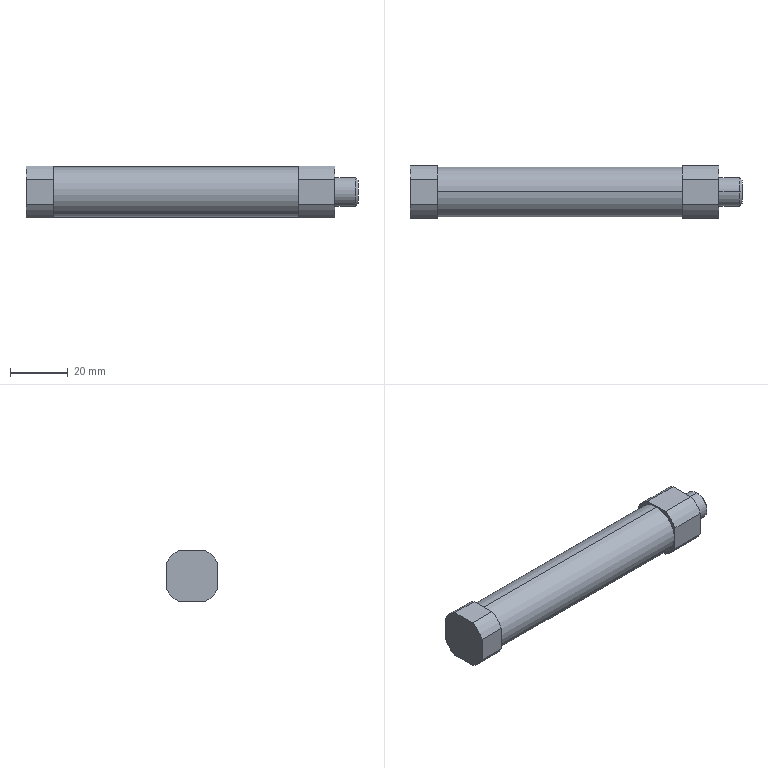Component | SolidWorks | A_CDJ2B16_60_B_0-1_CopyBody_A_CDJ2B16_60_B_0-1 | 1 solid | 40 faces | box 115 x 18 x 18 mm | volume 25719 mm3 | cylinder 18 | plane 16 | cone 6 | commonest cylinder face diameters 20 x8 4.13 x4 5.4 x2 17.4 x2 10 x2
STEP:
#1=COLOUR_RGB('',0.7922,0.8196,0.9333);
#2=FILL_AREA_STYLE_COLOUR('',#1);
#3=FILL_AREA_STYLE('',(#2));
#4=SURFACE_STYLE_FILL_AREA(#3);
#5=SURFACE_SIDE_STYLE('',(#4));
#6=SURFACE_STYLE_USAGE(.BOTH.,#5);
#7=PRESENTATION_STYLE_ASSIGNMENT((#6));
#8=CARTESIAN_POINT('',(-0.6587,0.8964,3.289));
#9=VERTEX_POINT('',#8);
#10=CARTESIAN_POINT('',(-0.6587,0.8964,3.076));
#11=VERTEX_POINT('',#10);
#12=CARTESIAN_POINT('',(-0.6587,0.8964,3.182));
#13=DIRECTION('',(1.,0.,0.));
#14=DIRECTION('',(0.,0.,-1.));
#15=AXIS2_PLACEMENT_3D('',#12,#13,#14);
#16=CIRCLE('',#15,0.1063);
#17=EDGE_CURVE('',#9,#11,#16,.T.);
#18=ORIENTED_EDGE('',*,*,#17,.F.);
#19=CARTESIAN_POINT('',(1.782,0.8964,3.289));
#20=VERTEX_POINT('',#19);
#21=CARTESIAN_POINT('',(-0.6587,0.8964,3.289));
#22=DIRECTION('',(1.,0.,0.));
#23=VECTOR('',#22,39.37);
#24=LINE('',#21,#23);
#25=EDGE_CURVE('',#9,#20,#24,.T.);
#26=ORIENTED_EDGE('',*,*,#25,.T.);
#27=CARTESIAN_POINT('',(1.782,0.8964,3.076));
#28=VERTEX_POINT('',#27);
#29=CARTESIAN_POINT('',(1.782,0.8964,3.182));
#30=DIRECTION('',(1.,0.,0.));
#31=DIRECTION('',(0.,0.,-1.));
#32=AXIS2_PLACEMENT_3D('',#29,#30,#31);
#33=CIRCLE('',#32,0.1063);
#34=EDGE_CURVE('',#20,#28,#33,.T.);
#35=ORIENTED_EDGE('',*,*,#34,.T.);
#36=CARTESIAN_POINT('',(-0.6587,0.8964,3.076));
#37=DIRECTION('',(1.,0.,0.));
#38=VECTOR('',#37,39.37);
#39=LINE('',#36,#38);
#40=EDGE_CURVE('',#11,#28,#39,.T.);
#41=ORIENTED_EDGE('',*,*,#40,.F.);
#42=EDGE_LOOP('',(#18,#26,#35,#41));
#43=FACE_OUTER_BOUND('',#42,.T.);
#44=CARTESIAN_POINT('',(-0.6587,0.8964,3.182));
#45=DIRECTION('',(1.,0.,0.));
#46=DIRECTION('',(0.,0.,-1.));
#47=AXIS2_PLACEMENT_3D('',#44,#45,#46);
#48=CYLINDRICAL_SURFACE('',#47,0.1063);
#49=ADVANCED_FACE('',(#43),#48,.F.);
#50=CARTESIAN_POINT('',(-2.63,1.133,3.182));
#51=VERTEX_POINT('',#50);
#52=CARTESIAN_POINT('',(-2.467,1.133,3.182));
#53=VERTEX_POINT('',#52);
#54=CARTESIAN_POINT('',(-2.548,1.133,3.182));
#55=DIRECTION('',(-0.,1.,-0.));
#56=DIRECTION('',(1.,0.,0.));
#57=AXIS2_PLACEMENT_3D('',#54,#55,#56);
#58=CIRCLE('',#57,0.0813);
#59=EDGE_CURVE('',#51,#53,#58,.T.);
#60=ORIENTED_EDGE('',*,*,#59,.F.);
#61=CARTESIAN_POINT('',(-2.63,1.231,3.182));
#62=VERTEX_POINT('',#61);
#63=CARTESIAN_POINT('',(-2.63,1.133,3.182));
#64=DIRECTION('',(-0.,1.,-0.));
#65=VECTOR('',#64,39.37);
#66=LINE('',#63,#65);
#67=EDGE_CURVE('',#51,#62,#66,.T.);
#68=ORIENTED_EDGE('',*,*,#67,.T.);
#69=CARTESIAN_POINT('',(-2.467,1.231,3.182));
#70=VERTEX_POINT('',#69);
#71=CARTESIAN_POINT('',(-2.548,1.231,3.182));
#72=DIRECTION('',(-0.,1.,-0.));
#73=DIRECTION('',(1.,0.,0.));
#74=AXIS2_PLACEMENT_3D('',#71,#72,#73);
#75=CIRCLE('',#74,0.0813);
#76=EDGE_CURVE('',#62,#70,#75,.T.);
#77=ORIENTED_EDGE('',*,*,#76,.T.);
#78=CARTESIAN_POINT('',(-2.467,1.133,3.182));
#79=DIRECTION('',(-0.,1.,-0.));
#80=VECTOR('',#79,39.37);
#81=LINE('',#78,#80);
#82=EDGE_CURVE('',#53,#70,#81,.T.);
#83=ORIENTED_EDGE('',*,*,#82,.F.);
#84=EDGE_LOOP('',(#60,#68,#77,#83));
#85=FACE_OUTER_BOUND('',#84,.T.);
#86=CARTESIAN_POINT('',(-2.548,1.133,3.182));
#87=DIRECTION('',(-0.,1.,-0.));
#88=DIRECTION('',(1.,0.,0.));
#89=AXIS2_PLACEMENT_3D('',#86,#87,#88);
#90=CYLINDRICAL_SURFACE('',#89,0.0813);
#91=ADVANCED_FACE('',(#85),#90,.F.);
#92=ORIENTED_EDGE('',*,*,#76,.F.);
#93=CARTESIAN_POINT('',(-2.649,1.251,3.182));
#94=VERTEX_POINT('',#93);
#95=CARTESIAN_POINT('',(-2.63,1.231,3.182));
#96=DIRECTION('',(-0.7071,0.7071,-0.));
#97=VECTOR('',#96,39.37);
#98=LINE('',#95,#97);
#99=EDGE_CURVE('',#62,#94,#98,.T.);
#100=ORIENTED_EDGE('',*,*,#99,.T.);
#101=CARTESIAN_POINT('',(-2.447,1.251,3.182));
#102=VERTEX_POINT('',#101);
#103=CARTESIAN_POINT('',(-2.548,1.251,3.182));
#104=DIRECTION('',(-0.,1.,-0.));
#105=DIRECTION('',(-1.,0.,0.));
#106=AXIS2_PLACEMENT_3D('',#103,#104,#105);
#107=CIRCLE('',#106,0.101);
#108=EDGE_CURVE('',#94,#102,#107,.T.);
#109=ORIENTED_EDGE('',*,*,#108,.T.);
#110=CARTESIAN_POINT('',(-2.467,1.231,3.182));
#111=DIRECTION('',(0.7071,0.7071,0.));
#112=VECTOR('',#111,39.37);
#113=LINE('',#110,#112);
#114=EDGE_CURVE('',#70,#102,#113,.T.);
#115=ORIENTED_EDGE('',*,*,#114,.F.);
#116=EDGE_LOOP('',(#92,#100,#109,#115));
#117=FACE_OUTER_BOUND('',#116,.T.);
#118=CARTESIAN_POINT('',(-2.548,1.231,3.182));
#119=DIRECTION('',(-0.,1.,-0.));
#120=DIRECTION('',(1.,0.,0.));
#121=AXIS2_PLACEMENT_3D('',#118,#119,#120);
#122=CONICAL_SURFACE('',#121,0.0813,0.7854);
#123=ADVANCED_FACE('',(#117),#122,.F.);
#124=CARTESIAN_POINT('',(1.071,1.133,3.182));
#125=VERTEX_POINT('',#124);
#126=CARTESIAN_POINT('',(1.234,1.133,3.182));
#127=VERTEX_POINT('',#126);
#128=CARTESIAN_POINT('',(1.152,1.133,3.182));
#129=DIRECTION('',(-0.,1.,-0.));
#130=DIRECTION('',(1.,0.,0.));
#131=AXIS2_PLACEMENT_3D('',#128,#129,#130);
#132=CIRCLE('',#131,0.0813);
#133=EDGE_CURVE('',#125,#127,#132,.T.);
#134=ORIENTED_EDGE('',*,*,#133,.F.);
#135=CARTESIAN_POINT('',(1.071,1.231,3.182));
#136=VERTEX_POINT('',#135);
#137=CARTESIAN_POINT('',(1.071,1.133,3.182));
#138=DIRECTION('',(-0.,1.,-0.));
#139=VECTOR('',#138,39.37);
#140=LINE('',#137,#139);
#141=EDGE_CURVE('',#125,#136,#140,.T.);
#142=ORIENTED_EDGE('',*,*,#141,.T.);
#143=CARTESIAN_POINT('',(1.234,1.231,3.182));
#144=VERTEX_POINT('',#143);
#145=CARTESIAN_POINT('',(1.152,1.231,3.182));
#146=DIRECTION('',(-0.,1.,-0.));
#147=DIRECTION('',(1.,0.,0.));
#148=AXIS2_PLACEMENT_3D('',#145,#146,#147);
#149=CIRCLE('',#148,0.0813);
#150=EDGE_CURVE('',#136,#144,#149,.T.);
#151=ORIENTED_EDGE('',*,*,#150,.T.);
#152=CARTESIAN_POINT('',(1.234,1.133,3.182));
#153=DIRECTION('',(-0.,1.,-0.));
#154=VECTOR('',#153,39.37);
#155=LINE('',#152,#154);
#156=EDGE_CURVE('',#127,#144,#155,.T.);
#157=ORIENTED_EDGE('',*,*,#156,.F.);
#158=EDGE_LOOP('',(#134,#142,#151,#157));
#159=FACE_OUTER_BOUND('',#158,.T.);
#160=CARTESIAN_POINT('',(1.152,1.133,3.182));
#161=DIRECTION('',(-0.,1.,-0.));
#162=DIRECTION('',(1.,0.,0.));
#163=AXIS2_PLACEMENT_3D('',#160,#161,#162);
#164=CYLINDRICAL_SURFACE('',#163,0.0813);
#165=ADVANCED_FACE('',(#159),#164,.F.);
#166=ORIENTED_EDGE('',*,*,#150,.F.);
#167=CARTESIAN_POINT('',(1.051,1.251,3.182));
#168=VERTEX_POINT('',#167);
#169=CARTESIAN_POINT('',(1.071,1.231,3.182));
#170=DIRECTION('',(-0.7071,0.7071,-0.));
#171=VECTOR('',#170,39.37);
#172=LINE('',#169,#171);
#173=EDGE_CURVE('',#136,#168,#172,.T.);
#174=ORIENTED_EDGE('',*,*,#173,.T.);
#175=CARTESIAN_POINT('',(1.253,1.251,3.182));
#176=VERTEX_POINT('',#175);
#177=CARTESIAN_POINT('',(1.152,1.251,3.182));
#178=DIRECTION('',(0.,-1.,0.));
#179=DIRECTION('',(1.,0.,0.));
#180=AXIS2_PLACEMENT_3D('',#177,#178,#179);
#181=CIRCLE('',#180,0.101);
#182=EDGE_CURVE('',#176,#168,#181,.T.);
#183=ORIENTED_EDGE('',*,*,#182,.F.);
#184=CARTESIAN_POINT('',(1.234,1.231,3.182));
#185=DIRECTION('',(0.7071,0.7071,0.));
#186=VECTOR('',#185,39.37);
#187=LINE('',#184,#186);
#188=EDGE_CURVE('',#144,#176,#187,.T.);
#189=ORIENTED_EDGE('',*,*,#188,.F.);
#190=EDGE_LOOP('',(#166,#174,#183,#189));
#191=FACE_OUTER_BOUND('',#190,.T.);
#192=CARTESIAN_POINT('',(1.152,1.231,3.182));
#193=DIRECTION('',(-0.,1.,-0.));
#194=DIRECTION('',(1.,0.,0.));
#195=AXIS2_PLACEMENT_3D('',#192,#193,#194);
#196=CONICAL_SURFACE('',#195,0.0813,0.7854);
#197=ADVANCED_FACE('',(#191),#196,.F.);
#198=CARTESIAN_POINT('',(-2.371,0.8964,2.84));
#199=VERTEX_POINT('',#198);
#200=CARTESIAN_POINT('',(-2.371,0.8964,3.525));
#201=VERTEX_POINT('',#200);
#202=CARTESIAN_POINT('',(-2.371,0.8964,3.182));
#203=DIRECTION('',(1.,0.,0.));
#204=DIRECTION('',(0.,0.,-1.));
#205=AXIS2_PLACEMENT_3D('',#202,#203,#204);
#206=CIRCLE('',#205,0.3425);
#207=EDGE_CURVE('',#199,#201,#206,.T.);
#208=ORIENTED_EDGE('',*,*,#207,.T.);
#209=CARTESIAN_POINT('',(0.9752,0.8964,3.525));
#210=VERTEX_POINT('',#209);
#211=CARTESIAN_POINT('',(-2.735,0.8964,3.525));
#212=DIRECTION('',(1.,0.,0.));
#213=VECTOR('',#212,39.37);
#214=LINE('',#211,#213);
#215=EDGE_CURVE('',#201,#210,#214,.T.);
#216=ORIENTED_EDGE('',*,*,#215,.T.);
#217=CARTESIAN_POINT('',(0.9752,0.8964,2.84));
#218=VERTEX_POINT('',#217);
#219=CARTESIAN_POINT('',(0.9752,0.8964,3.182));
#220=DIRECTION('',(1.,0.,0.));
#221=DIRECTION('',(0.,0.,-1.));
#222=AXIS2_PLACEMENT_3D('',#219,#220,#221);
#223=CIRCLE('',#222,0.3425);
#224=EDGE_CURVE('',#218,#210,#223,.T.);
#225=ORIENTED_EDGE('',*,*,#224,.F.);
#226=CARTESIAN_POINT('',(-2.735,0.8964,2.84));
#227=DIRECTION('',(1.,0.,0.));
#228=VECTOR('',#227,39.37);
#229=LINE('',#226,#228);
#230=EDGE_CURVE('',#199,#218,#229,.T.);
#231=ORIENTED_EDGE('',*,*,#230,.F.);
#232=EDGE_LOOP('',(#208,#216,#225,#231));
#233=FACE_OUTER_BOUND('',#232,.T.);
#234=CARTESIAN_POINT('',(-2.735,0.8964,3.182));
#235=DIRECTION('',(1.,0.,0.));
#236=DIRECTION('',(0.,0.,-1.));
#237=AXIS2_PLACEMENT_3D('',#234,#235,#236);
#238=CYLINDRICAL_SURFACE('',#237,0.3425);
#239=ADVANCED_FACE('',(#233),#238,.T.);
#240=CARTESIAN_POINT('',(1.467,0.8964,2.985));
#241=VERTEX_POINT('',#240);
#242=CARTESIAN_POINT('',(1.467,0.8964,3.379));
#243=VERTEX_POINT('',#242);
#244=CARTESIAN_POINT('',(1.467,0.8964,3.182));
#245=DIRECTION('',(1.,0.,0.));
#246=DIRECTION('',(0.,0.,-1.));
#247=AXIS2_PLACEMENT_3D('',#244,#245,#246);
#248=CIRCLE('',#247,0.1969);
#249=EDGE_CURVE('',#241,#243,#248,.T.);
#250=ORIENTED_EDGE('',*,*,#249,.T.);
#251=CARTESIAN_POINT('',(1.746,0.8964,3.379));
#252=VERTEX_POINT('',#251);
#253=CARTESIAN_POINT('',(-2.735,0.8964,3.379));
#254=DIRECTION('',(1.,0.,0.));
#255=VECTOR('',#254,39.37);
#256=LINE('',#253,#255);
#257=EDGE_CURVE('',#243,#252,#256,.T.);
#258=ORIENTED_EDGE('',*,*,#257,.T.);
#259=CARTESIAN_POINT('',(1.746,0.8964,2.985));
#260=VERTEX_POINT('',#259);
#261=CARTESIAN_POINT('',(1.746,0.8964,3.182));
#262=DIRECTION('',(1.,0.,0.));
#263=DIRECTION('',(0.,0.,-1.));
#264=AXIS2_PLACEMENT_3D('',#261,#262,#263);
#265=CIRCLE('',#264,0.1969);
#266=EDGE_CURVE('',#260,#252,#265,.T.);
#267=ORIENTED_EDGE('',*,*,#266,.F.);
#268=CARTESIAN_POINT('',(-2.735,0.8964,2.985));
#269=DIRECTION('',(1.,0.,0.));
#270=VECTOR('',#269,39.37);
#271=LINE('',#268,#270);
#272=EDGE_CURVE('',#241,#260,#271,.T.);
#273=ORIENTED_EDGE('',*,*,#272,.F.);
#274=EDGE_LOOP('',(#250,#258,#267,#273));
#275=FACE_OUTER_BOUND('',#274,.T.);
#276=CARTESIAN_POINT('',(-2.735,0.8964,3.182));
#277=DIRECTION('',(1.,0.,0.));
#278=DIRECTION('',(0.,0.,-1.));
#279=AXIS2_PLACEMENT_3D('',#276,#277,#278);
#280=CYLINDRICAL_SURFACE('',#279,0.1969);
#281=ADVANCED_FACE('',(#275),#280,.T.);
#282=CARTESIAN_POINT('',(1.782,0.8964,3.022));
#283=VERTEX_POINT('',#282);
#284=CARTESIAN_POINT('',(1.782,0.8964,3.343));
#285=VERTEX_POINT('',#284);
#286=CARTESIAN_POINT('',(1.782,0.8964,3.182));
#287=DIRECTION('',(1.,0.,0.));
#288=DIRECTION('',(0.,0.,-1.));
#289=AXIS2_PLACEMENT_3D('',#286,#287,#288);
#290=CIRCLE('',#289,0.1606);
#291=EDGE_CURVE('',#283,#285,#290,.T.);
#292=ORIENTED_EDGE('',*,*,#291,.F.);
#293=CARTESIAN_POINT('',(1.746,0.8964,2.985));
#294=DIRECTION('',(-0.7071,0.,-0.7071));
#295=VECTOR('',#294,39.37);
#296=LINE('',#293,#295);
#297=EDGE_CURVE('',#283,#260,#296,.T.);
#298=ORIENTED_EDGE('',*,*,#297,.T.);
#299=ORIENTED_EDGE('',*,*,#266,.T.);
#300=CARTESIAN_POINT('',(1.746,0.8964,3.379));
#301=DIRECTION('',(-0.7071,-0.,0.7071));
#302=VECTOR('',#301,39.37);
#303=LINE('',#300,#302);
#304=EDGE_CURVE('',#285,#252,#303,.T.);
#305=ORIENTED_EDGE('',*,*,#304,.F.);
#306=EDGE_LOOP('',(#292,#298,#299,#305));
#307=FACE_OUTER_BOUND('',#306,.T.);
#308=CARTESIAN_POINT('',(1.746,0.8964,3.182));
#309=DIRECTION('',(-1.,-0.,-0.));
#310=DIRECTION('',(0.,0.,1.));
#311=AXIS2_PLACEMENT_3D('',#308,#309,#310);
#312=CONICAL_SURFACE('',#311,0.1969,0.7854);
#313=ADVANCED_FACE('',(#307),#312,.T.);
#314=CARTESIAN_POINT('',(-2.745,1.251,3.011));
#315=VERTEX_POINT('',#314);
#316=CARTESIAN_POINT('',(-2.745,1.251,3.354));
#317=VERTEX_POINT('',#316);
#318=CARTESIAN_POINT('',(-2.745,1.251,3.011));
#319=DIRECTION('',(-0.,0.,1.));
#320=VECTOR('',#319,39.37);
#321=LINE('',#318,#320);
#322=EDGE_CURVE('',#315,#317,#321,.T.);
#323=ORIENTED_EDGE('',*,*,#322,.T.);
#324=CARTESIAN_POINT('',(-2.371,1.251,3.354));
#325=VERTEX_POINT('',#324);
#326=CARTESIAN_POINT('',(-2.371,1.251,3.354));
#327=DIRECTION('',(-1.,-0.,-0.));
#328=VECTOR('',#327,39.37);
#329=LINE('',#326,#328);
#330=EDGE_CURVE('',#325,#317,#329,.T.);
#331=ORIENTED_EDGE('',*,*,#330,.F.);
#332=CARTESIAN_POINT('',(-2.371,1.251,3.011));
#333=VERTEX_POINT('',#332);
#334=CARTESIAN_POINT('',(-2.371,1.251,3.011));
#335=DIRECTION('',(-0.,0.,1.));
#336=VECTOR('',#335,39.37);
#337=LINE('',#334,#336);
#338=EDGE_CURVE('',#333,#325,#337,.T.);
#339=ORIENTED_EDGE('',*,*,#338,.F.);
#340=CARTESIAN_POINT('',(-2.371,1.251,3.011));
#341=DIRECTION('',(-1.,-0.,-0.));
#342=VECTOR('',#341,39.37);
#343=LINE('',#340,#342);
#344=EDGE_CURVE('',#333,#315,#343,.T.);
#345=ORIENTED_EDGE('',*,*,#344,.T.);
#346=EDGE_LOOP('',(#323,#331,#339,#345));
#347=FACE_OUTER_BOUND('',#346,.T.);
#348=CARTESIAN_POINT('',(-2.548,1.251,3.182));
#349=DIRECTION('',(-0.,1.,-0.));
#350=DIRECTION('',(-1.,0.,0.));
#351=AXIS2_PLACEMENT_3D('',#348,#349,#350);
#352=CIRCLE('',#351,0.101);
#353=EDGE_CURVE('',#102,#94,#352,.T.);
#354=ORIENTED_EDGE('',*,*,#353,.F.);
#355=ORIENTED_EDGE('',*,*,#108,.F.);
#356=EDGE_LOOP('',(#354,#355));
#357=FACE_BOUND('',#356,.T.);
#358=CARTESIAN_POINT('',(-2.371,1.251,3.011));
#359=DIRECTION('',(0.,-1.,0.));
#360=DIRECTION('',(-1.,-0.,-0.));
#361=AXIS2_PLACEMENT_3D('',#358,#359,#360);
#362=PLANE('',#361);
#363=ADVANCED_FACE('',(#347,#357),#362,.F.);
#364=CARTESIAN_POINT('',(1.467,1.251,3.011));
#365=VERTEX_POINT('',#364);
#366=CARTESIAN_POINT('',(1.467,1.251,3.354));
#367=VERTEX_POINT('',#366);
#368=CARTESIAN_POINT('',(1.467,1.251,3.011));
#369=DIRECTION('',(-0.,0.,1.));
#370=VECTOR('',#369,39.37);
#371=LINE('',#368,#370);
#372=EDGE_CURVE('',#365,#367,#371,.T.);
#373=ORIENTED_EDGE('',*,*,#372,.F.);
#374=CARTESIAN_POINT('',(0.9752,1.251,3.011));
#375=VERTEX_POINT('',#374);
#376=CARTESIAN_POINT('',(0.9752,1.251,3.011));
#377=DIRECTION('',(1.,0.,0.));
#378=VECTOR('',#377,39.37);
#379=LINE('',#376,#378);
#380=EDGE_CURVE('',#375,#365,#379,.T.);
#381=ORIENTED_EDGE('',*,*,#380,.F.);
#382=CARTESIAN_POINT('',(0.9752,1.251,3.354));
#383=VERTEX_POINT('',#382);
#384=CARTESIAN_POINT('',(0.9752,1.251,3.011));
#385=DIRECTION('',(-0.,0.,1.));
#386=VECTOR('',#385,39.37);
#387=LINE('',#384,#386);
#388=EDGE_CURVE('',#375,#383,#387,.T.);
#389=ORIENTED_EDGE('',*,*,#388,.T.);
#390=CARTESIAN_POINT('',(0.9752,1.251,3.354));
#391=DIRECTION('',(1.,0.,0.));
#392=VECTOR('',#391,39.37);
#393=LINE('',#390,#392);
#394=EDGE_CURVE('',#383,#367,#393,.T.);
#395=ORIENTED_EDGE('',*,*,#394,.T.);
#396=EDGE_LOOP('',(#373,#381,#389,#395));
#397=FACE_OUTER_BOUND('',#396,.T.);
#398=ORIENTED_EDGE('',*,*,#182,.T.);
#399=CARTESIAN_POINT('',(1.152,1.251,3.182));
#400=DIRECTION('',(0.,-1.,0.));
#401=DIRECTION('',(1.,0.,0.));
#402=AXIS2_PLACEMENT_3D('',#399,#400,#401);
#403=CIRCLE('',#402,0.101);
#404=EDGE_CURVE('',#168,#176,#403,.T.);
#405=ORIENTED_EDGE('',*,*,#404,.T.);
#406=EDGE_LOOP('',(#398,#405));
#407=FACE_BOUND('',#406,.T.);
#408=CARTESIAN_POINT('',(0.9752,1.251,3.011));
#409=DIRECTION('',(-0.,1.,-0.));
#410=DIRECTION('',(1.,0.,0.));
#411=AXIS2_PLACEMENT_3D('',#408,#409,#410);
#412=PLANE('',#411);
#413=ADVANCED_FACE('',(#397,#407),#412,.T.);
#414=CARTESIAN_POINT('',(1.782,0.8964,3.182));
#415=DIRECTION('',(1.,0.,0.));
#416=DIRECTION('',(0.,0.,-1.));
#417=AXIS2_PLACEMENT_3D('',#414,#415,#416);
#418=CIRCLE('',#417,0.1063);
#419=EDGE_CURVE('',#28,#20,#418,.T.);
#420=ORIENTED_EDGE('',*,*,#419,.F.);
#421=ORIENTED_EDGE('',*,*,#34,.F.);
#422=EDGE_LOOP('',(#420,#421));
#423=FACE_BOUND('',#422,.T.);
#424=CARTESIAN_POINT('',(1.782,0.8964,3.182));
#425=DIRECTION('',(1.,0.,0.));
#426=DIRECTION('',(0.,0.,-1.));
#427=AXIS2_PLACEMENT_3D('',#424,#425,#426);
#428=CIRCLE('',#427,0.1606);
#429=EDGE_CURVE('',#285,#283,#428,.T.);
#430=ORIENTED_EDGE('',*,*,#429,.T.);
#431=ORIENTED_EDGE('',*,*,#291,.T.);
#432=EDGE_LOOP('',(#430,#431));
#433=FACE_OUTER_BOUND('',#432,.T.);
#434=CARTESIAN_POINT('',(1.782,0.8964,3.182));
#435=DIRECTION('',(-1.,-0.,-0.));
#436=DIRECTION('',(-0.,0.,1.));
#437=AXIS2_PLACEMENT_3D('',#434,#435,#436);
#438=PLANE('',#437);
#439=ADVANCED_FACE('',(#423,#433),#438,.F.);
#440=ORIENTED_EDGE('',*,*,#297,.F.);
#441=ORIENTED_EDGE('',*,*,#429,.F.);
#442=ORIENTED_EDGE('',*,*,#304,.T.);
#443=CARTESIAN_POINT('',(1.746,0.8964,3.182));
#444=DIRECTION('',(1.,0.,0.));
#445=DIRECTION('',(0.,0.,-1.));
#446=AXIS2_PLACEMENT_3D('',#443,#444,#445);
#447=CIRCLE('',#446,0.1969);
#448=EDGE_CURVE('',#252,#260,#447,.T.);
#449=ORIENTED_EDGE('',*,*,#448,.T.);
#450=EDGE_LOOP('',(#440,#441,#442,#449));
#451=FACE_OUTER_BOUND('',#450,.T.);
#452=CARTESIAN_POINT('',(1.746,0.8964,3.182));
#453=DIRECTION('',(-1.,-0.,-0.));
#454=DIRECTION('',(0.,0.,1.));
#455=AXIS2_PLACEMENT_3D('',#452,#453,#454);
#456=CONICAL_SURFACE('',#455,0.1969,0.7854);
#457=ADVANCED_FACE('',(#451),#456,.T.);
#458=ORIENTED_EDGE('',*,*,#257,.F.);
#459=CARTESIAN_POINT('',(1.467,0.8964,3.182));
#460=DIRECTION('',(1.,0.,0.));
#461=DIRECTION('',(0.,0.,-1.));
#462=AXIS2_PLACEMENT_3D('',#459,#460,#461);
#463=CIRCLE('',#462,0.1969);
#464=EDGE_CURVE('',#243,#241,#463,.T.);
#465=ORIENTED_EDGE('',*,*,#464,.T.);
#466=ORIENTED_EDGE('',*,*,#272,.T.);
#467=ORIENTED_EDGE('',*,*,#448,.F.);
#468=EDGE_LOOP('',(#458,#465,#466,#467));
#469=FACE_OUTER_BOUND('',#468,.T.);
#470=CARTESIAN_POINT('',(-2.735,0.8964,3.182));
#471=DIRECTION('',(1.,0.,0.));
#472=DIRECTION('',(0.,0.,-1.));
#473=AXIS2_PLACEMENT_3D('',#470,#471,#472);
#474=CYLINDRICAL_SURFACE('',#473,0.1969);
#475=ADVANCED_FACE('',(#469),#474,.T.);
#476=CARTESIAN_POINT('',(1.467,0.7248,3.537));
#477=VERTEX_POINT('',#476);
#478=CARTESIAN_POINT('',(1.467,0.5421,3.354));
#479=VERTEX_POINT('',#478);
#480=CARTESIAN_POINT('',(1.467,0.8964,3.182));
#481=DIRECTION('',(1.,0.,0.));
#482=DIRECTION('',(0.,0.,-1.));
#483=AXIS2_PLACEMENT_3D('',#480,#481,#482);
#484=CIRCLE('',#483,0.3937);
#485=EDGE_CURVE('',#477,#479,#484,.T.);
#486=ORIENTED_EDGE('',*,*,#485,.T.);
#487=CARTESIAN_POINT('',(1.467,0.5421,3.011));
#488=VERTEX_POINT('',#487);
#489=CARTESIAN_POINT('',(1.467,0.5421,3.354));
#490=DIRECTION('',(0.,-0.,-1.));
#491=VECTOR('',#490,39.37);
#492=LINE('',#489,#491);
#493=EDGE_CURVE('',#479,#488,#492,.T.);
#494=ORIENTED_EDGE('',*,*,#493,.T.);
#495=CARTESIAN_POINT('',(1.467,0.7248,2.828));
#496=VERTEX_POINT('',#495);
#497=CARTESIAN_POINT('',(1.467,0.8964,3.182));
#498=DIRECTION('',(1.,0.,0.));
#499=DIRECTION('',(0.,0.,-1.));
#500=AXIS2_PLACEMENT_3D('',#497,#498,#499);
#501=CIRCLE('',#500,0.3937);
#502=EDGE_CURVE('',#488,#496,#501,.T.);
#503=ORIENTED_EDGE('',*,*,#502,.T.);
#504=CARTESIAN_POINT('',(1.467,1.068,2.828));
#505=VERTEX_POINT('',#504);
#506=CARTESIAN_POINT('',(1.467,0.7248,2.828));
#507=DIRECTION('',(-0.,1.,-0.));
#508=VECTOR('',#507,39.37);
#509=LINE('',#506,#508);
#510=EDGE_CURVE('',#496,#505,#509,.T.);
#511=ORIENTED_EDGE('',*,*,#510,.T.);
#512=CARTESIAN_POINT('',(1.467,0.8964,3.182));
#513=DIRECTION('',(1.,0.,0.));
#514=DIRECTION('',(0.,0.,-1.));
#515=AXIS2_PLACEMENT_3D('',#512,#513,#514);
#516=CIRCLE('',#515,0.3937);
#517=EDGE_CURVE('',#505,#365,#516,.T.);
#518=ORIENTED_EDGE('',*,*,#517,.T.);
#519=ORIENTED_EDGE('',*,*,#372,.T.);
#520=CARTESIAN_POINT('',(1.467,1.068,3.537));
#521=VERTEX_POINT('',#520);
#522=CARTESIAN_POINT('',(1.467,0.8964,3.182));
#523=DIRECTION('',(1.,0.,0.));
#524=DIRECTION('',(0.,0.,-1.));
#525=AXIS2_PLACEMENT_3D('',#522,#523,#524);
#526=CIRCLE('',#525,0.3937);
#527=EDGE_CURVE('',#367,#521,#526,.T.);
#528=ORIENTED_EDGE('',*,*,#527,.T.);
#529=CARTESIAN_POINT('',(1.467,1.068,3.537));
#530=DIRECTION('',(0.,-1.,0.));
#531=VECTOR('',#530,39.37);
#532=LINE('',#529,#531);
#533=EDGE_CURVE('',#521,#477,#532,.T.);
#534=ORIENTED_EDGE('',*,*,#533,.T.);
#535=EDGE_LOOP('',(#486,#494,#503,#511,#518,#519,#528,#534));
#536=FACE_OUTER_BOUND('',#535,.T.);
#537=ORIENTED_EDGE('',*,*,#249,.F.);
#538=ORIENTED_EDGE('',*,*,#464,.F.);
#539=EDGE_LOOP('',(#537,#538));
#540=FACE_BOUND('',#539,.T.);
#541=CARTESIAN_POINT('',(1.467,0.8964,3.182));
#542=DIRECTION('',(1.,0.,0.));
#543=DIRECTION('',(0.,-0.,-1.));
#544=AXIS2_PLACEMENT_3D('',#541,#542,#543);
#545=PLANE('',#544);
#546=ADVANCED_FACE('',(#536,#540),#545,.T.);
#547=CARTESIAN_POINT('',(0.9752,0.7248,3.537));
#548=VERTEX_POINT('',#547);
#549=CARTESIAN_POINT('',(0.9752,0.5421,3.354));
#550=VERTEX_POINT('',#549);
#551=CARTESIAN_POINT('',(0.9752,0.8964,3.182));
#552=DIRECTION('',(1.,0.,0.));
#553=DIRECTION('',(0.,0.,-1.));
#554=AXIS2_PLACEMENT_3D('',#551,#552,#553);
#555=CIRCLE('',#554,0.3937);
#556=EDGE_CURVE('',#548,#550,#555,.T.);
#557=ORIENTED_EDGE('',*,*,#556,.F.);
#558=CARTESIAN_POINT('',(0.9752,1.068,3.537));
#559=VERTEX_POINT('',#558);
#560=CARTESIAN_POINT('',(0.9752,1.068,3.537));
#561=DIRECTION('',(0.,-1.,0.));
#562=VECTOR('',#561,39.37);
#563=LINE('',#560,#562);
#564=EDGE_CURVE('',#559,#548,#563,.T.);
#565=ORIENTED_EDGE('',*,*,#564,.F.);
#566=CARTESIAN_POINT('',(0.9752,0.8964,3.182));
#567=DIRECTION('',(1.,0.,0.));
#568=DIRECTION('',(0.,0.,-1.));
#569=AXIS2_PLACEMENT_3D('',#566,#567,#568);
#570=CIRCLE('',#569,0.3937);
#571=EDGE_CURVE('',#383,#559,#570,.T.);
#572=ORIENTED_EDGE('',*,*,#571,.F.);
#573=ORIENTED_EDGE('',*,*,#388,.F.);
#574=CARTESIAN_POINT('',(0.9752,1.068,2.828));
#575=VERTEX_POINT('',#574);
#576=CARTESIAN_POINT('',(0.9752,0.8964,3.182));
#577=DIRECTION('',(1.,0.,0.));
#578=DIRECTION('',(0.,0.,-1.));
#579=AXIS2_PLACEMENT_3D('',#576,#577,#578);
#580=CIRCLE('',#579,0.3937);
#581=EDGE_CURVE('',#575,#375,#580,.T.);
#582=ORIENTED_EDGE('',*,*,#581,.F.);
#583=CARTESIAN_POINT('',(0.9752,0.7248,2.828));
#584=VERTEX_POINT('',#583);
#585=CARTESIAN_POINT('',(0.9752,0.7248,2.828));
#586=DIRECTION('',(-0.,1.,-0.));
#587=VECTOR('',#586,39.37);
#588=LINE('',#585,#587);
#589=EDGE_CURVE('',#584,#575,#588,.T.);
#590=ORIENTED_EDGE('',*,*,#589,.F.);
#591=CARTESIAN_POINT('',(0.9752,0.5421,3.011));
#592=VERTEX_POINT('',#591);
#593=CARTESIAN_POINT('',(0.9752,0.8964,3.182));
#594=DIRECTION('',(1.,0.,0.));
#595=DIRECTION('',(0.,0.,-1.));
#596=AXIS2_PLACEMENT_3D('',#593,#594,#595);
#597=CIRCLE('',#596,0.3937);
#598=EDGE_CURVE('',#592,#584,#597,.T.);
#599=ORIENTED_EDGE('',*,*,#598,.F.);
#600=CARTESIAN_POINT('',(0.9752,0.5421,3.354));
#601=DIRECTION('',(0.,-0.,-1.));
#602=VECTOR('',#601,39.37);
#603=LINE('',#600,#602);
#604=EDGE_CURVE('',#550,#592,#603,.T.);
#605=ORIENTED_EDGE('',*,*,#604,.F.);
#606=EDGE_LOOP('',(#557,#565,#572,#573,#582,#590,#599,#605));
#607=FACE_OUTER_BOUND('',#606,.T.);
#608=ORIENTED_EDGE('',*,*,#224,.T.);
#609=CARTESIAN_POINT('',(0.9752,0.8964,3.182));
#610=DIRECTION('',(1.,0.,0.));
#611=DIRECTION('',(0.,0.,-1.));
#612=AXIS2_PLACEMENT_3D('',#609,#610,#611);
#613=CIRCLE('',#612,0.3425);
#614=EDGE_CURVE('',#210,#218,#613,.T.);
#615=ORIENTED_EDGE('',*,*,#614,.T.);
#616=EDGE_LOOP('',(#608,#615));
#617=FACE_BOUND('',#616,.T.);
#618=CARTESIAN_POINT('',(0.9752,0.8964,3.182));
#619=DIRECTION('',(1.,0.,0.));
#620=DIRECTION('',(0.,-0.,-1.));
#621=AXIS2_PLACEMENT_3D('',#618,#619,#620);
#622=PLANE('',#621);
#623=ADVANCED_FACE('',(#607,#617),#622,.F.);
#624=ORIENTED_EDGE('',*,*,#485,.F.);
#625=CARTESIAN_POINT('',(0.9752,0.7248,3.537));
#626=DIRECTION('',(1.,0.,0.));
#627=VECTOR('',#626,39.37);
#628=LINE('',#625,#627);
#629=EDGE_CURVE('',#548,#477,#628,.T.);
#630=ORIENTED_EDGE('',*,*,#629,.F.);
#631=ORIENTED_EDGE('',*,*,#556,.T.);
#632=CARTESIAN_POINT('',(0.9752,0.5421,3.354));
#633=DIRECTION('',(1.,0.,0.));
#634=VECTOR('',#633,39.37);
#635=LINE('',#632,#634);
#636=EDGE_CURVE('',#550,#479,#635,.T.);
#637=ORIENTED_EDGE('',*,*,#636,.T.);
#638=EDGE_LOOP('',(#624,#630,#631,#637));
#639=FACE_OUTER_BOUND('',#638,.T.);
#640=CARTESIAN_POINT('',(0.9752,0.8964,3.182));
#641=DIRECTION('',(1.,0.,0.));
#642=DIRECTION('',(0.,0.,-1.));
#643=AXIS2_PLACEMENT_3D('',#640,#641,#642);
#644=CYLINDRICAL_SURFACE('',#643,0.3937);
#645=ADVANCED_FACE('',(#639),#644,.T.);
#646=ORIENTED_EDGE('',*,*,#533,.F.);
#647=CARTESIAN_POINT('',(0.9752,1.068,3.537));
#648=DIRECTION('',(1.,0.,0.));
#649=VECTOR('',#648,39.37);
#650=LINE('',#647,#649);
#651=EDGE_CURVE('',#559,#521,#650,.T.);
#652=ORIENTED_EDGE('',*,*,#651,.F.);
#653=ORIENTED_EDGE('',*,*,#564,.T.);
#654=ORIENTED_EDGE('',*,*,#629,.T.);
#655=EDGE_LOOP('',(#646,#652,#653,#654));
#656=FACE_OUTER_BOUND('',#655,.T.);
#657=CARTESIAN_POINT('',(0.9752,1.068,3.537));
#658=DIRECTION('',(-0.,0.,1.));
#659=DIRECTION('',(1.,0.,0.));
#660=AXIS2_PLACEMENT_3D('',#657,#658,#659);
#661=PLANE('',#660);
#662=ADVANCED_FACE('',(#656),#661,.T.);
#663=ORIENTED_EDGE('',*,*,#527,.F.);
#664=ORIENTED_EDGE('',*,*,#394,.F.);
#665=ORIENTED_EDGE('',*,*,#571,.T.);
#666=ORIENTED_EDGE('',*,*,#651,.T.);
#667=EDGE_LOOP('',(#663,#664,#665,#666));
#668=FACE_OUTER_BOUND('',#667,.T.);
#669=CARTESIAN_POINT('',(0.9752,0.8964,3.182));
#670=DIRECTION('',(1.,0.,0.));
#671=DIRECTION('',(0.,0.,-1.));
#672=AXIS2_PLACEMENT_3D('',#669,#670,#671);
#673=CYLINDRICAL_SURFACE('',#672,0.3937);
#674=ADVANCED_FACE('',(#668),#673,.T.);
#675=ORIENTED_EDGE('',*,*,#517,.F.);
#676=CARTESIAN_POINT('',(0.9752,1.068,2.828));
#677=DIRECTION('',(1.,0.,0.));
#678=VECTOR('',#677,39.37);
#679=LINE('',#676,#678);
#680=EDGE_CURVE('',#575,#505,#679,.T.);
#681=ORIENTED_EDGE('',*,*,#680,.F.);
#682=ORIENTED_EDGE('',*,*,#581,.T.);
#683=ORIENTED_EDGE('',*,*,#380,.T.);
#684=EDGE_LOOP('',(#675,#681,#682,#683));
#685=FACE_OUTER_BOUND('',#684,.T.);
#686=CARTESIAN_POINT('',(0.9752,0.8964,3.182));
#687=DIRECTION('',(1.,0.,0.));
#688=DIRECTION('',(0.,0.,-1.));
#689=AXIS2_PLACEMENT_3D('',#686,#687,#688);
#690=CYLINDRICAL_SURFACE('',#689,0.3937);
#691=ADVANCED_FACE('',(#685),#690,.T.);
#692=ORIENTED_EDGE('',*,*,#510,.F.);
#693=CARTESIAN_POINT('',(0.9752,0.7248,2.828));
#694=DIRECTION('',(1.,0.,0.));
#695=VECTOR('',#694,39.37);
#696=LINE('',#693,#695);
#697=EDGE_CURVE('',#584,#496,#696,.T.);
#698=ORIENTED_EDGE('',*,*,#697,.F.);
#699=ORIENTED_EDGE('',*,*,#589,.T.);
#700=ORIENTED_EDGE('',*,*,#680,.T.);
#701=EDGE_LOOP('',(#692,#698,#699,#700));
#702=FACE_OUTER_BOUND('',#701,.T.);
#703=CARTESIAN_POINT('',(0.9752,0.7248,2.828));
#704=DIRECTION('',(0.,-0.,-1.));
#705=DIRECTION('',(-1.,-0.,-0.));
#706=AXIS2_PLACEMENT_3D('',#703,#704,#705);
#707=PLANE('',#706);
#708=ADVANCED_FACE('',(#702),#707,.T.);
#709=ORIENTED_EDGE('',*,*,#502,.F.);
#710=CARTESIAN_POINT('',(0.9752,0.5421,3.011));
#711=DIRECTION('',(1.,0.,0.));
#712=VECTOR('',#711,39.37);
#713=LINE('',#710,#712);
#714=EDGE_CURVE('',#592,#488,#713,.T.);
#715=ORIENTED_EDGE('',*,*,#714,.F.);
#716=ORIENTED_EDGE('',*,*,#598,.T.);
#717=ORIENTED_EDGE('',*,*,#697,.T.);
#718=EDGE_LOOP('',(#709,#715,#716,#717));
#719=FACE_OUTER_BOUND('',#718,.T.);
#720=CARTESIAN_POINT('',(0.9752,0.8964,3.182));
#721=DIRECTION('',(1.,0.,0.));
#722=DIRECTION('',(0.,0.,-1.));
#723=AXIS2_PLACEMENT_3D('',#720,#721,#722);
#724=CYLINDRICAL_SURFACE('',#723,0.3937);
#725=ADVANCED_FACE('',(#719),#724,.T.);
#726=ORIENTED_EDGE('',*,*,#493,.F.);
#727=ORIENTED_EDGE('',*,*,#636,.F.);
#728=ORIENTED_EDGE('',*,*,#604,.T.);
#729=ORIENTED_EDGE('',*,*,#714,.T.);
#730=EDGE_LOOP('',(#726,#727,#728,#729));
#731=FACE_OUTER_BOUND('',#730,.T.);
#732=CARTESIAN_POINT('',(0.9752,0.5421,3.354));
#733=DIRECTION('',(0.,-1.,0.));
#734=DIRECTION('',(-1.,-0.,-0.));
#735=AXIS2_PLACEMENT_3D('',#732,#733,#734);
#736=PLANE('',#735);
#737=ADVANCED_FACE('',(#731),#736,.T.);
#738=ORIENTED_EDGE('',*,*,#215,.F.);
#739=CARTESIAN_POINT('',(-2.371,0.8964,3.182));
#740=DIRECTION('',(1.,0.,0.));
#741=DIRECTION('',(0.,0.,-1.));
#742=AXIS2_PLACEMENT_3D('',#739,#740,#741);
#743=CIRCLE('',#742,0.3425);
#744=EDGE_CURVE('',#201,#199,#743,.T.);
#745=ORIENTED_EDGE('',*,*,#744,.T.);
#746=ORIENTED_EDGE('',*,*,#230,.T.);
#747=ORIENTED_EDGE('',*,*,#614,.F.);
#748=EDGE_LOOP('',(#738,#745,#746,#747));
#749=FACE_OUTER_BOUND('',#748,.T.);
#750=CARTESIAN_POINT('',(-2.735,0.8964,3.182));
#751=DIRECTION('',(1.,0.,0.));
#752=DIRECTION('',(0.,0.,-1.));
#753=AXIS2_PLACEMENT_3D('',#750,#751,#752);
#754=CYLINDRICAL_SURFACE('',#753,0.3425);
#755=ADVANCED_FACE('',(#749),#754,.T.);
#756=CARTESIAN_POINT('',(-2.371,0.7248,3.537));
#757=VERTEX_POINT('',#756);
#758=CARTESIAN_POINT('',(-2.371,0.5421,3.354));
#759=VERTEX_POINT('',#758);
#760=CARTESIAN_POINT('',(-2.371,0.8964,3.182));
#761=DIRECTION('',(1.,0.,0.));
#762=DIRECTION('',(0.,0.,-1.));
#763=AXIS2_PLACEMENT_3D('',#760,#761,#762);
#764=CIRCLE('',#763,0.3937);
#765=EDGE_CURVE('',#757,#759,#764,.T.);
#766=ORIENTED_EDGE('',*,*,#765,.T.);
#767=CARTESIAN_POINT('',(-2.371,0.5421,3.011));
#768=VERTEX_POINT('',#767);
#769=CARTESIAN_POINT('',(-2.371,0.5421,3.354));
#770=DIRECTION('',(0.,-0.,-1.));
#771=VECTOR('',#770,39.37);
#772=LINE('',#769,#771);
#773=EDGE_CURVE('',#759,#768,#772,.T.);
#774=ORIENTED_EDGE('',*,*,#773,.T.);
#775=CARTESIAN_POINT('',(-2.371,0.7248,2.828));
#776=VERTEX_POINT('',#775);
#777=CARTESIAN_POINT('',(-2.371,0.8964,3.182));
#778=DIRECTION('',(1.,0.,0.));
#779=DIRECTION('',(0.,0.,-1.));
#780=AXIS2_PLACEMENT_3D('',#777,#778,#779);
#781=CIRCLE('',#780,0.3937);
#782=EDGE_CURVE('',#768,#776,#781,.T.);
#783=ORIENTED_EDGE('',*,*,#782,.T.);
#784=CARTESIAN_POINT('',(-2.371,1.068,2.828));
#785=VERTEX_POINT('',#784);
#786=CARTESIAN_POINT('',(-2.371,0.7248,2.828));
#787=DIRECTION('',(-0.,1.,-0.));
#788=VECTOR('',#787,39.37);
#789=LINE('',#786,#788);
#790=EDGE_CURVE('',#776,#785,#789,.T.);
#791=ORIENTED_EDGE('',*,*,#790,.T.);
#792=CARTESIAN_POINT('',(-2.371,0.8964,3.182));
#793=DIRECTION('',(1.,0.,0.));
#794=DIRECTION('',(0.,0.,-1.));
#795=AXIS2_PLACEMENT_3D('',#792,#793,#794);
#796=CIRCLE('',#795,0.3937);
#797=EDGE_CURVE('',#785,#333,#796,.T.);
#798=ORIENTED_EDGE('',*,*,#797,.T.);
#799=ORIENTED_EDGE('',*,*,#338,.T.);
#800=CARTESIAN_POINT('',(-2.371,1.068,3.537));
#801=VERTEX_POINT('',#800);
#802=CARTESIAN_POINT('',(-2.371,0.8964,3.182));
#803=DIRECTION('',(1.,0.,0.));
#804=DIRECTION('',(0.,0.,-1.));
#805=AXIS2_PLACEMENT_3D('',#802,#803,#804);
#806=CIRCLE('',#805,0.3937);
#807=EDGE_CURVE('',#325,#801,#806,.T.);
#808=ORIENTED_EDGE('',*,*,#807,.T.);
#809=CARTESIAN_POINT('',(-2.371,1.068,3.537));
#810=DIRECTION('',(0.,-1.,0.));
#811=VECTOR('',#810,39.37);
#812=LINE('',#809,#811);
#813=EDGE_CURVE('',#801,#757,#812,.T.);
#814=ORIENTED_EDGE('',*,*,#813,.T.);
#815=EDGE_LOOP('',(#766,#774,#783,#791,#798,#799,#808,#814));
#816=FACE_OUTER_BOUND('',#815,.T.);
#817=ORIENTED_EDGE('',*,*,#207,.F.);
#818=ORIENTED_EDGE('',*,*,#744,.F.);
#819=EDGE_LOOP('',(#817,#818));
#820=FACE_BOUND('',#819,.T.);
#821=CARTESIAN_POINT('',(-2.371,0.8964,3.182));
#822=DIRECTION('',(1.,0.,0.));
#823=DIRECTION('',(0.,-0.,-1.));
#824=AXIS2_PLACEMENT_3D('',#821,#822,#823);
#825=PLANE('',#824);
#826=ADVANCED_FACE('',(#816,#820),#825,.T.);
#827=CARTESIAN_POINT('',(-2.745,0.7248,3.537));
#828=VERTEX_POINT('',#827);
#829=CARTESIAN_POINT('',(-2.745,0.5421,3.354));
#830=VERTEX_POINT('',#829);
#831=CARTESIAN_POINT('',(-2.745,0.8964,3.182));
#832=DIRECTION('',(1.,0.,0.));
#833=DIRECTION('',(0.,0.,-1.));
#834=AXIS2_PLACEMENT_3D('',#831,#832,#833);
#835=CIRCLE('',#834,0.3937);
#836=EDGE_CURVE('',#828,#830,#835,.T.);
#837=ORIENTED_EDGE('',*,*,#836,.T.);
#838=CARTESIAN_POINT('',(-2.371,0.5421,3.354));
#839=DIRECTION('',(-1.,-0.,-0.));
#840=VECTOR('',#839,39.37);
#841=LINE('',#838,#840);
#842=EDGE_CURVE('',#759,#830,#841,.T.);
#843=ORIENTED_EDGE('',*,*,#842,.F.);
#844=ORIENTED_EDGE('',*,*,#765,.F.);
#845=CARTESIAN_POINT('',(-2.371,0.7248,3.537));
#846=DIRECTION('',(-1.,-0.,-0.));
#847=VECTOR('',#846,39.37);
#848=LINE('',#845,#847);
#849=EDGE_CURVE('',#757,#828,#848,.T.);
#850=ORIENTED_EDGE('',*,*,#849,.T.);
#851=EDGE_LOOP('',(#837,#843,#844,#850));
#852=FACE_OUTER_BOUND('',#851,.T.);
#853=CARTESIAN_POINT('',(-2.371,0.8964,3.182));
#854=DIRECTION('',(-1.,-0.,-0.));
#855=DIRECTION('',(0.,0.,1.));
#856=AXIS2_PLACEMENT_3D('',#853,#854,#855);
#857=CYLINDRICAL_SURFACE('',#856,0.3937);
#858=ADVANCED_FACE('',(#852),#857,.T.);
#859=CARTESIAN_POINT('',(-2.745,0.5421,3.011));
#860=VERTEX_POINT('',#859);
#861=CARTESIAN_POINT('',(-2.745,0.5421,3.354));
#862=DIRECTION('',(0.,-0.,-1.));
#863=VECTOR('',#862,39.37);
#864=LINE('',#861,#863);
#865=EDGE_CURVE('',#830,#860,#864,.T.);
#866=ORIENTED_EDGE('',*,*,#865,.T.);
#867=CARTESIAN_POINT('',(-2.371,0.5421,3.011));
#868=DIRECTION('',(-1.,-0.,-0.));
#869=VECTOR('',#868,39.37);
#870=LINE('',#867,#869);
#871=EDGE_CURVE('',#768,#860,#870,.T.);
#872=ORIENTED_EDGE('',*,*,#871,.F.);
#873=ORIENTED_EDGE('',*,*,#773,.F.);
#874=ORIENTED_EDGE('',*,*,#842,.T.);
#875=EDGE_LOOP('',(#866,#872,#873,#874));
#876=FACE_OUTER_BOUND('',#875,.T.);
#877=CARTESIAN_POINT('',(-2.371,0.5421,3.354));
#878=DIRECTION('',(-0.,1.,-0.));
#879=DIRECTION('',(1.,0.,0.));
#880=AXIS2_PLACEMENT_3D('',#877,#878,#879);
#881=PLANE('',#880);
#882=ADVANCED_FACE('',(#876),#881,.F.);
#883=CARTESIAN_POINT('',(-2.745,0.7248,2.828));
#884=VERTEX_POINT('',#883);
#885=CARTESIAN_POINT('',(-2.745,0.8964,3.182));
#886=DIRECTION('',(1.,0.,0.));
#887=DIRECTION('',(0.,0.,-1.));
#888=AXIS2_PLACEMENT_3D('',#885,#886,#887);
#889=CIRCLE('',#888,0.3937);
#890=EDGE_CURVE('',#860,#884,#889,.T.);
#891=ORIENTED_EDGE('',*,*,#890,.T.);
#892=CARTESIAN_POINT('',(-2.371,0.7248,2.828));
#893=DIRECTION('',(-1.,-0.,-0.));
#894=VECTOR('',#893,39.37);
#895=LINE('',#892,#894);
#896=EDGE_CURVE('',#776,#884,#895,.T.);
#897=ORIENTED_EDGE('',*,*,#896,.F.);
#898=ORIENTED_EDGE('',*,*,#782,.F.);
#899=ORIENTED_EDGE('',*,*,#871,.T.);
#900=EDGE_LOOP('',(#891,#897,#898,#899));
#901=FACE_OUTER_BOUND('',#900,.T.);
#902=CARTESIAN_POINT('',(-2.371,0.8964,3.182));
#903=DIRECTION('',(-1.,-0.,-0.));
#904=DIRECTION('',(0.,0.,1.));
#905=AXIS2_PLACEMENT_3D('',#902,#903,#904);
#906=CYLINDRICAL_SURFACE('',#905,0.3937);
#907=ADVANCED_FACE('',(#901),#906,.T.);
#908=CARTESIAN_POINT('',(-2.745,1.068,2.828));
#909=VERTEX_POINT('',#908);
#910=CARTESIAN_POINT('',(-2.745,0.7248,2.828));
#911=DIRECTION('',(-0.,1.,-0.));
#912=VECTOR('',#911,39.37);
#913=LINE('',#910,#912);
#914=EDGE_CURVE('',#884,#909,#913,.T.);
#915=ORIENTED_EDGE('',*,*,#914,.T.);
#916=CARTESIAN_POINT('',(-2.371,1.068,2.828));
#917=DIRECTION('',(-1.,-0.,-0.));
#918=VECTOR('',#917,39.37);
#919=LINE('',#916,#918);
#920=EDGE_CURVE('',#785,#909,#919,.T.);
#921=ORIENTED_EDGE('',*,*,#920,.F.);
#922=ORIENTED_EDGE('',*,*,#790,.F.);
#923=ORIENTED_EDGE('',*,*,#896,.T.);
#924=EDGE_LOOP('',(#915,#921,#922,#923));
#925=FACE_OUTER_BOUND('',#924,.T.);
#926=CARTESIAN_POINT('',(-2.371,0.7248,2.828));
#927=DIRECTION('',(-0.,0.,1.));
#928=DIRECTION('',(1.,0.,0.));
#929=AXIS2_PLACEMENT_3D('',#926,#927,#928);
#930=PLANE('',#929);
#931=ADVANCED_FACE('',(#925),#930,.F.);
#932=CARTESIAN_POINT('',(-2.745,0.8964,3.182));
#933=DIRECTION('',(1.,0.,0.));
#934=DIRECTION('',(0.,0.,-1.));
#935=AXIS2_PLACEMENT_3D('',#932,#933,#934);
#936=CIRCLE('',#935,0.3937);
#937=EDGE_CURVE('',#909,#315,#936,.T.);
#938=ORIENTED_EDGE('',*,*,#937,.T.);
#939=ORIENTED_EDGE('',*,*,#344,.F.);
#940=ORIENTED_EDGE('',*,*,#797,.F.);
#941=ORIENTED_EDGE('',*,*,#920,.T.);
#942=EDGE_LOOP('',(#938,#939,#940,#941));
#943=FACE_OUTER_BOUND('',#942,.T.);
#944=CARTESIAN_POINT('',(-2.371,0.8964,3.182));
#945=DIRECTION('',(-1.,-0.,-0.));
#946=DIRECTION('',(0.,0.,1.));
#947=AXIS2_PLACEMENT_3D('',#944,#945,#946);
#948=CYLINDRICAL_SURFACE('',#947,0.3937);
#949=ADVANCED_FACE('',(#943),#948,.T.);
#950=CARTESIAN_POINT('',(-2.745,1.068,3.537));
#951=VERTEX_POINT('',#950);
#952=CARTESIAN_POINT('',(-2.745,0.8964,3.182));
#953=DIRECTION('',(1.,0.,0.));
#954=DIRECTION('',(0.,0.,-1.));
#955=AXIS2_PLACEMENT_3D('',#952,#953,#954);
#956=CIRCLE('',#955,0.3937);
#957=EDGE_CURVE('',#317,#951,#956,.T.);
#958=ORIENTED_EDGE('',*,*,#957,.T.);
#959=CARTESIAN_POINT('',(-2.371,1.068,3.537));
#960=DIRECTION('',(-1.,-0.,-0.));
#961=VECTOR('',#960,39.37);
#962=LINE('',#959,#961);
#963=EDGE_CURVE('',#801,#951,#962,.T.);
#964=ORIENTED_EDGE('',*,*,#963,.F.);
#965=ORIENTED_EDGE('',*,*,#807,.F.);
#966=ORIENTED_EDGE('',*,*,#330,.T.);
#967=EDGE_LOOP('',(#958,#964,#965,#966));
#968=FACE_OUTER_BOUND('',#967,.T.);
#969=CARTESIAN_POINT('',(-2.371,0.8964,3.182));
#970=DIRECTION('',(-1.,-0.,-0.));
#971=DIRECTION('',(0.,0.,1.));
#972=AXIS2_PLACEMENT_3D('',#969,#970,#971);
#973=CYLINDRICAL_SURFACE('',#972,0.3937);
#974=ADVANCED_FACE('',(#968),#973,.T.);
#975=CARTESIAN_POINT('',(-2.745,1.068,3.537));
#976=DIRECTION('',(0.,-1.,0.));
#977=VECTOR('',#976,39.37);
#978=LINE('',#975,#977);
#979=EDGE_CURVE('',#951,#828,#978,.T.);
#980=ORIENTED_EDGE('',*,*,#979,.T.);
#981=ORIENTED_EDGE('',*,*,#849,.F.);
#982=ORIENTED_EDGE('',*,*,#813,.F.);
#983=ORIENTED_EDGE('',*,*,#963,.T.);
#984=EDGE_LOOP('',(#980,#981,#982,#983));
#985=FACE_OUTER_BOUND('',#984,.T.);
#986=CARTESIAN_POINT('',(-2.371,1.068,3.537));
#987=DIRECTION('',(0.,-0.,-1.));
#988=DIRECTION('',(-1.,-0.,-0.));
#989=AXIS2_PLACEMENT_3D('',#986,#987,#988);
#990=PLANE('',#989);
#991=ADVANCED_FACE('',(#985),#990,.F.);
#992=ORIENTED_EDGE('',*,*,#836,.F.);
#993=ORIENTED_EDGE('',*,*,#979,.F.);
#994=ORIENTED_EDGE('',*,*,#957,.F.);
#995=ORIENTED_EDGE('',*,*,#322,.F.);
#996=ORIENTED_EDGE('',*,*,#937,.F.);
#997=ORIENTED_EDGE('',*,*,#914,.F.);
#998=ORIENTED_EDGE('',*,*,#890,.F.);
#999=ORIENTED_EDGE('',*,*,#865,.F.);
#1000=EDGE_LOOP('',(#992,#993,#994,#995,#996,#997,#998,#999));
#1001=FACE_OUTER_BOUND('',#1000,.T.);
#1002=CARTESIAN_POINT('',(-2.745,0.8964,3.182));
#1003=DIRECTION('',(1.,0.,0.));
#1004=DIRECTION('',(0.,-0.,-1.));
#1005=AXIS2_PLACEMENT_3D('',#1002,#1003,#1004);
#1006=PLANE('',#1005);
#1007=ADVANCED_FACE('',(#1001),#1006,.F.);
#1008=ORIENTED_EDGE('',*,*,#173,.F.);
#1009=CARTESIAN_POINT('',(1.152,1.231,3.182));
#1010=DIRECTION('',(-0.,1.,-0.));
#1011=DIRECTION('',(1.,0.,0.));
#1012=AXIS2_PLACEMENT_3D('',#1009,#1010,#1011);
#1013=CIRCLE('',#1012,0.0813);
#1014=EDGE_CURVE('',#144,#136,#1013,.T.);
#1015=ORIENTED_EDGE('',*,*,#1014,.F.);
#1016=ORIENTED_EDGE('',*,*,#188,.T.);
#1017=ORIENTED_EDGE('',*,*,#404,.F.);
#1018=EDGE_LOOP('',(#1008,#1015,#1016,#1017));
#1019=FACE_OUTER_BOUND('',#1018,.T.);
#1020=CARTESIAN_POINT('',(1.152,1.231,3.182));
#1021=DIRECTION('',(-0.,1.,-0.));
#1022=DIRECTION('',(1.,0.,0.));
#1023=AXIS2_PLACEMENT_3D('',#1020,#1021,#1022);
#1024=CONICAL_SURFACE('',#1023,0.0813,0.7854);
#1025=ADVANCED_FACE('',(#1019),#1024,.F.);
#1026=ORIENTED_EDGE('',*,*,#141,.F.);
#1027=CARTESIAN_POINT('',(1.152,1.133,3.182));
#1028=DIRECTION('',(-0.,1.,-0.));
#1029=DIRECTION('',(1.,0.,0.));
#1030=AXIS2_PLACEMENT_3D('',#1027,#1028,#1029);
#1031=CIRCLE('',#1030,0.0813);
#1032=EDGE_CURVE('',#127,#125,#1031,.T.);
#1033=ORIENTED_EDGE('',*,*,#1032,.F.);
#1034=ORIENTED_EDGE('',*,*,#156,.T.);
#1035=ORIENTED_EDGE('',*,*,#1014,.T.);
#1036=EDGE_LOOP('',(#1026,#1033,#1034,#1035));
#1037=FACE_OUTER_BOUND('',#1036,.T.);
#1038=CARTESIAN_POINT('',(1.152,1.133,3.182));
#1039=DIRECTION('',(-0.,1.,-0.));
#1040=DIRECTION('',(1.,0.,0.));
#1041=AXIS2_PLACEMENT_3D('',#1038,#1039,#1040);
#1042=CYLINDRICAL_SURFACE('',#1041,0.0813);
#1043=ADVANCED_FACE('',(#1037),#1042,.F.);
#1044=ORIENTED_EDGE('',*,*,#1032,.T.);
#1045=ORIENTED_EDGE('',*,*,#133,.T.);
#1046=EDGE_LOOP('',(#1044,#1045));
#1047=FACE_OUTER_BOUND('',#1046,.T.);
#1048=CARTESIAN_POINT('',(1.152,1.133,3.101));
#1049=DIRECTION('',(-0.,1.,-0.));
#1050=DIRECTION('',(1.,0.,0.));
#1051=AXIS2_PLACEMENT_3D('',#1048,#1049,#1050);
#1052=PLANE('',#1051);
#1053=ADVANCED_FACE('',(#1047),#1052,.T.);
#1054=ORIENTED_EDGE('',*,*,#99,.F.);
#1055=CARTESIAN_POINT('',(-2.548,1.231,3.182));
#1056=DIRECTION('',(-0.,1.,-0.));
#1057=DIRECTION('',(1.,0.,0.));
#1058=AXIS2_PLACEMENT_3D('',#1055,#1056,#1057);
#1059=CIRCLE('',#1058,0.0813);
#1060=EDGE_CURVE('',#70,#62,#1059,.T.);
#1061=ORIENTED_EDGE('',*,*,#1060,.F.);
#1062=ORIENTED_EDGE('',*,*,#114,.T.);
#1063=ORIENTED_EDGE('',*,*,#353,.T.);
#1064=EDGE_LOOP('',(#1054,#1061,#1062,#1063));
#1065=FACE_OUTER_BOUND('',#1064,.T.);
#1066=CARTESIAN_POINT('',(-2.548,1.231,3.182));
#1067=DIRECTION('',(-0.,1.,-0.));
#1068=DIRECTION('',(1.,0.,0.));
#1069=AXIS2_PLACEMENT_3D('',#1066,#1067,#1068);
#1070=CONICAL_SURFACE('',#1069,0.0813,0.7854);
#1071=ADVANCED_FACE('',(#1065),#1070,.F.);
#1072=ORIENTED_EDGE('',*,*,#67,.F.);
#1073=CARTESIAN_POINT('',(-2.548,1.133,3.182));
#1074=DIRECTION('',(-0.,1.,-0.));
#1075=DIRECTION('',(1.,0.,0.));
#1076=AXIS2_PLACEMENT_3D('',#1073,#1074,#1075);
#1077=CIRCLE('',#1076,0.0813);
#1078=EDGE_CURVE('',#53,#51,#1077,.T.);
#1079=ORIENTED_EDGE('',*,*,#1078,.F.);
#1080=ORIENTED_EDGE('',*,*,#82,.T.);
#1081=ORIENTED_EDGE('',*,*,#1060,.T.);
#1082=EDGE_LOOP('',(#1072,#1079,#1080,#1081));
#1083=FACE_OUTER_BOUND('',#1082,.T.);
#1084=CARTESIAN_POINT('',(-2.548,1.133,3.182));
#1085=DIRECTION('',(-0.,1.,-0.));
#1086=DIRECTION('',(1.,0.,0.));
#1087=AXIS2_PLACEMENT_3D('',#1084,#1085,#1086);
#1088=CYLINDRICAL_SURFACE('',#1087,0.0813);
#1089=ADVANCED_FACE('',(#1083),#1088,.F.);
#1090=ORIENTED_EDGE('',*,*,#1078,.T.);
#1091=ORIENTED_EDGE('',*,*,#59,.T.);
#1092=EDGE_LOOP('',(#1090,#1091));
#1093=FACE_OUTER_BOUND('',#1092,.T.);
#1094=CARTESIAN_POINT('',(-2.548,1.133,3.101));
#1095=DIRECTION('',(-0.,1.,-0.));
#1096=DIRECTION('',(1.,0.,0.));
#1097=AXIS2_PLACEMENT_3D('',#1094,#1095,#1096);
#1098=PLANE('',#1097);
#1099=ADVANCED_FACE('',(#1093),#1098,.T.);
#1100=ORIENTED_EDGE('',*,*,#25,.F.);
#1101=CARTESIAN_POINT('',(-0.6587,0.8964,3.182));
#1102=DIRECTION('',(1.,0.,0.));
#1103=DIRECTION('',(0.,0.,-1.));
#1104=AXIS2_PLACEMENT_3D('',#1101,#1102,#1103);
#1105=CIRCLE('',#1104,0.1063);
#1106=EDGE_CURVE('',#11,#9,#1105,.T.);
#1107=ORIENTED_EDGE('',*,*,#1106,.F.);
#1108=ORIENTED_EDGE('',*,*,#40,.T.);
#1109=ORIENTED_EDGE('',*,*,#419,.T.);
#1110=EDGE_LOOP('',(#1100,#1107,#1108,#1109));
#1111=FACE_OUTER_BOUND('',#1110,.T.);
#1112=CARTESIAN_POINT('',(-0.6587,0.8964,3.182));
#1113=DIRECTION('',(1.,0.,0.));
#1114=DIRECTION('',(0.,0.,-1.));
#1115=AXIS2_PLACEMENT_3D('',#1112,#1113,#1114);
#1116=CYLINDRICAL_SURFACE('',#1115,0.1063);
#1117=ADVANCED_FACE('',(#1111),#1116,.F.);
#1118=ORIENTED_EDGE('',*,*,#1106,.T.);
#1119=ORIENTED_EDGE('',*,*,#17,.T.);
#1120=EDGE_LOOP('',(#1118,#1119));
#1121=FACE_OUTER_BOUND('',#1120,.T.);
#1122=CARTESIAN_POINT('',(-0.6587,0.8964,3.182));
#1123=DIRECTION('',(1.,0.,0.));
#1124=DIRECTION('',(0.,-0.,-1.));
#1125=AXIS2_PLACEMENT_3D('',#1122,#1123,#1124);
#1126=PLANE('',#1125);
#1127=ADVANCED_FACE('',(#1121),#1126,.T.);
#1128=CLOSED_SHELL('',(#49,#91,#123,#165,#197,#239,#281,#313,#363,#413,#439,#457,#475,#546,#623,#645,#662,#674,#691,#708,#725,#737,#755,#826,#858,#882,#907,#931,#949,#974,#991,#1007,#1025,#1043,#1053,#1071,#1089,#1099,#1117,#1127));
#1129=MANIFOLD_SOLID_BREP('',#1128);
#1130=STYLED_ITEM('',(#7),#1129);
#1131=(LENGTH_UNIT()NAMED_UNIT(*)SI_UNIT($,.METRE.));
#1132=LENGTH_MEASURE_WITH_UNIT(LENGTH_MEASURE(0.0254),#1131);
#1133=DIMENSIONAL_EXPONENTS(1.,0.,0.,0.,0.,0.,0.);
#1134=(CONVERSION_BASED_UNIT('',#1132)LENGTH_UNIT()NAMED_UNIT(#1133));
#1135=UNCERTAINTY_MEASURE_WITH_UNIT(LENGTH_MEASURE(0.00001),#1134,'','');
#1136=(NAMED_UNIT(*)PLANE_ANGLE_UNIT()SI_UNIT($,.RADIAN.));
#1137=(NAMED_UNIT(*)SI_UNIT($,.STERADIAN.)SOLID_ANGLE_UNIT());
#1138=(GEOMETRIC_REPRESENTATION_CONTEXT(3)GLOBAL_UNCERTAINTY_ASSIGNED_CONTEXT((#1135))GLOBAL_UNIT_ASSIGNED_CONTEXT((#1134,#1136,#1137))REPRESENTATION_CONTEXT('',''));
#1139=MECHANICAL_DESIGN_GEOMETRIC_PRESENTATION_REPRESENTATION('',(#1130),#1138);
#1140=PRESENTATION_LAYER_ASSIGNMENT('','',(#1130));
#1141=CARTESIAN_POINT('',(0.,0.,0.));
#1142=DIRECTION('',(0.,0.,1.));
#1143=DIRECTION('',(1.,0.,0.));
#1144=AXIS2_PLACEMENT_3D('',#1141,#1142,#1143);
#1145=(LENGTH_UNIT()NAMED_UNIT(*)SI_UNIT($,.METRE.));
#1146=LENGTH_MEASURE_WITH_UNIT(LENGTH_MEASURE(0.0254),#1145);
#1147=DIMENSIONAL_EXPONENTS(1.,0.,0.,0.,0.,0.,0.);
#1148=(CONVERSION_BASED_UNIT('',#1146)LENGTH_UNIT()NAMED_UNIT(#1147));
#1149=UNCERTAINTY_MEASURE_WITH_UNIT(LENGTH_MEASURE(0.00001),#1148,'','');
#1150=(NAMED_UNIT(*)PLANE_ANGLE_UNIT()SI_UNIT($,.RADIAN.));
#1151=(NAMED_UNIT(*)SI_UNIT($,.STERADIAN.)SOLID_ANGLE_UNIT());
#1152=(GEOMETRIC_REPRESENTATION_CONTEXT(3)GLOBAL_UNCERTAINTY_ASSIGNED_CONTEXT((#1149))GLOBAL_UNIT_ASSIGNED_CONTEXT((#1148,#1150,#1151))REPRESENTATION_CONTEXT('',''));
#1153=ADVANCED_BREP_SHAPE_REPRESENTATION('',(#1129,#1144),#1152);